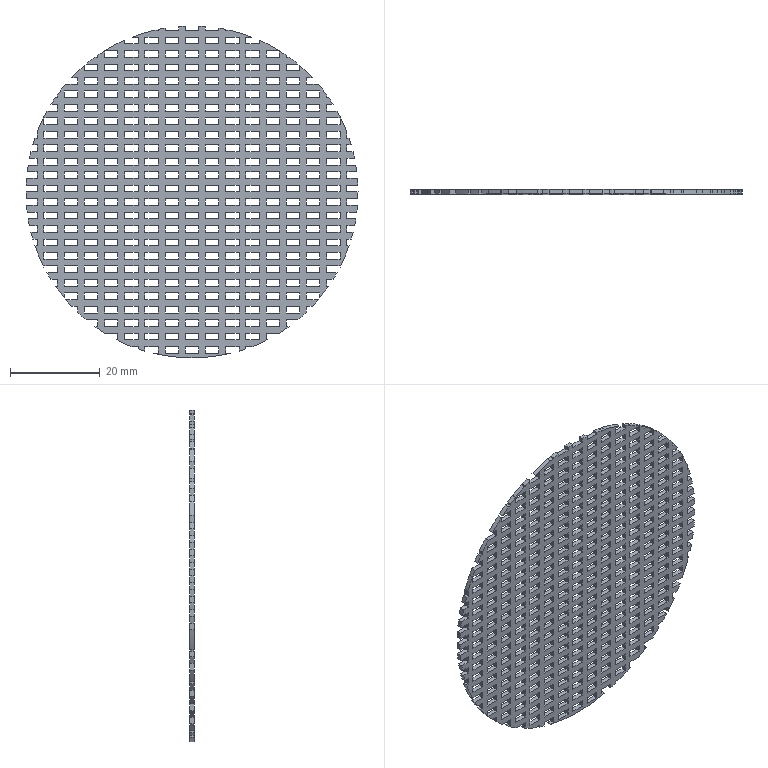Component | SolidWorks | Filtre moteur-1 | 1 solid | 1380 faces | box 74 x 1 x 73.97 mm | volume 2865 mm3 | plane 1325 | cylinder 55 | commonest cylinder face diameters 74 x55